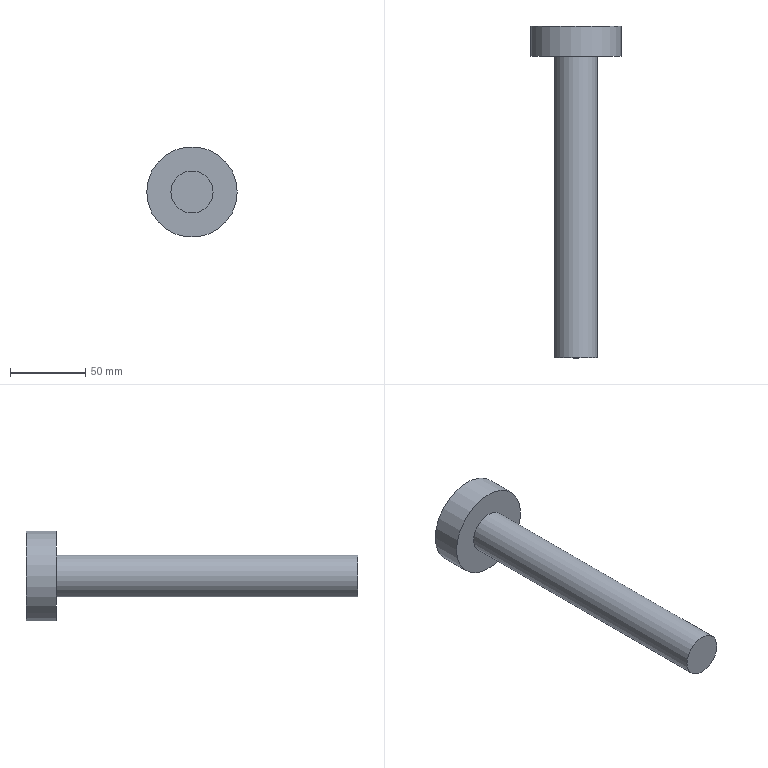Component | NX | PIN_2 | 1 solid | 5 faces | box 60 x 220 x 60 mm | volume 179699 mm3 | plane 3 | cylinder 2 | commonest cylinder face diameters 28 x1 60 x1
STEP:
#1=CARTESIAN_POINT('',(0.,0.,0.));
#2=DIRECTION('',(0.,0.,1.));
#3=DIRECTION('',(1.,0.,0.));
#4=AXIS2_PLACEMENT_3D('',#1,#2,#3);
#5=CARTESIAN_POINT('',(191.055,38.,82.998));
#6=VERTEX_POINT('',#5);
#7=CARTESIAN_POINT('',(177.055,38.,82.998));
#8=DIRECTION('',(0.,1.,0.));
#9=DIRECTION('',(1.,0.,0.));
#10=AXIS2_PLACEMENT_3D('',#7,#8,#9);
#11=CIRCLE('',#10,14.);
#12=CARTESIAN_POINT('',(177.055,38.,82.998));
#13=DIRECTION('',(0.,-1.,0.));
#14=DIRECTION('',(-1.,0.,0.));
#15=AXIS2_PLACEMENT_3D('',#12,#13,#14);
#16=PLANE('',#15);
#17=CARTESIAN_POINT('',(-14.,0.));
#18=CARTESIAN_POINT('',(-14.,24.249));
#19=CARTESIAN_POINT('',(7.,12.124));
#20=CARTESIAN_POINT('',(28.,0.));
#21=CARTESIAN_POINT('',(7.,-12.124));
#22=CARTESIAN_POINT('',(-14.,-24.249));
#23=CARTESIAN_POINT('',(-14.,0.));
#24=(BOUNDED_CURVE()B_SPLINE_CURVE(2,(#17,#18,#19,#20,#21,#22,#23),.UNSPECIFIED.,.T.,.F.)B_SPLINE_CURVE_WITH_KNOTS((1,2,2,2,2,1),(-2.094,0.,2.094,4.189,6.283,8.378),.UNSPECIFIED.)CURVE()GEOMETRIC_REPRESENTATION_ITEM()RATIONAL_B_SPLINE_CURVE((1.,0.5,1.,0.5,1.,0.5,1.))REPRESENTATION_ITEM(''));
#25=(GEOMETRIC_REPRESENTATION_CONTEXT(2)PARAMETRIC_REPRESENTATION_CONTEXT()REPRESENTATION_CONTEXT('',''));
#26=DEFINITIONAL_REPRESENTATION('',(#24),#25);
#27=PCURVE('',#16,#26);
#28=CARTESIAN_POINT('',(177.055,38.,82.998));
#29=DIRECTION('',(0.,1.,0.));
#30=DIRECTION('',(1.,0.,0.));
#31=AXIS2_PLACEMENT_3D('',#28,#29,#30);
#32=CYLINDRICAL_SURFACE('',#31,14.);
#33=CARTESIAN_POINT('',(0.,0.));
#34=DIRECTION('',(1.,0.));
#35=VECTOR('',#34,1.);
#36=LINE('',#33,#35);
#37=(GEOMETRIC_REPRESENTATION_CONTEXT(2)PARAMETRIC_REPRESENTATION_CONTEXT()REPRESENTATION_CONTEXT('',''));
#38=DEFINITIONAL_REPRESENTATION('',(#36),#37);
#39=PCURVE('',#32,#38);
#40=SURFACE_CURVE('',#11,(#27,#39),.PCURVE_S1.);
#41=EDGE_CURVE('',#6,#6,#40,.T.);
#42=ORIENTED_EDGE('',*,*,#41,.F.);
#43=EDGE_LOOP('',(#42));
#44=FACE_BOUND('',#43,.T.);
#45=ADVANCED_FACE('',(#44),#16,.T.);
#46=CARTESIAN_POINT('',(191.055,238.,82.998));
#47=VERTEX_POINT('',#46);
#48=CARTESIAN_POINT('',(177.055,238.,82.998));
#49=DIRECTION('',(0.,-1.,0.));
#50=DIRECTION('',(1.,0.,0.));
#51=AXIS2_PLACEMENT_3D('',#48,#49,#50);
#52=CIRCLE('',#51,14.);
#53=CARTESIAN_POINT('',(6.283,200.));
#54=DIRECTION('',(-1.,0.));
#55=VECTOR('',#54,1.);
#56=LINE('',#53,#55);
#57=(GEOMETRIC_REPRESENTATION_CONTEXT(2)PARAMETRIC_REPRESENTATION_CONTEXT()REPRESENTATION_CONTEXT('',''));
#58=DEFINITIONAL_REPRESENTATION('',(#56),#57);
#59=PCURVE('',#32,#58);
#60=CARTESIAN_POINT('',(177.055,238.,82.998));
#61=DIRECTION('',(0.,-1.,0.));
#62=DIRECTION('',(-1.,0.,0.));
#63=AXIS2_PLACEMENT_3D('',#60,#61,#62);
#64=PLANE('',#63);
#65=CARTESIAN_POINT('',(0.,0.));
#66=DIRECTION('',(-1.,0.));
#67=AXIS2_PLACEMENT_2D('',#65,#66);
#68=CIRCLE('',#67,14.);
#69=(GEOMETRIC_REPRESENTATION_CONTEXT(2)PARAMETRIC_REPRESENTATION_CONTEXT()REPRESENTATION_CONTEXT('',''));
#70=DEFINITIONAL_REPRESENTATION('',(#68),#69);
#71=PCURVE('',#64,#70);
#72=SURFACE_CURVE('',#52,(#59,#71),.PCURVE_S1.);
#73=EDGE_CURVE('',#47,#47,#72,.T.);
#74=ORIENTED_EDGE('',*,*,#73,.T.);
#75=CARTESIAN_POINT('',(191.055,38.,82.998));
#76=CARTESIAN_POINT('',(191.055,238.,82.998));
#77=B_SPLINE_CURVE_WITH_KNOTS('',1,(#75,#76),.UNSPECIFIED.,.F.,.F.,(2,2),(0.,200.),.PIECEWISE_BEZIER_KNOTS.);
#78=CARTESIAN_POINT('',(0.,0.));
#79=DIRECTION('',(0.,1.));
#80=VECTOR('',#79,1.);
#81=LINE('',#78,#80);
#82=(GEOMETRIC_REPRESENTATION_CONTEXT(2)PARAMETRIC_REPRESENTATION_CONTEXT()REPRESENTATION_CONTEXT('',''));
#83=DEFINITIONAL_REPRESENTATION('',(#81),#82);
#84=PCURVE('',#32,#83);
#85=CARTESIAN_POINT('',(6.283,0.));
#86=DIRECTION('',(0.,1.));
#87=VECTOR('',#86,1.);
#88=LINE('',#85,#87);
#89=(GEOMETRIC_REPRESENTATION_CONTEXT(2)PARAMETRIC_REPRESENTATION_CONTEXT()REPRESENTATION_CONTEXT('',''));
#90=DEFINITIONAL_REPRESENTATION('',(#88),#89);
#91=PCURVE('',#32,#90);
#92=SEAM_CURVE('',#77,(#84,#91),.PCURVE_S1.);
#93=EDGE_CURVE('',#6,#47,#92,.T.);
#94=ORIENTED_EDGE('',*,*,#93,.F.);
#95=ORIENTED_EDGE('',*,*,#41,.T.);
#96=ORIENTED_EDGE('',*,*,#93,.T.);
#97=EDGE_LOOP('',(#74,#94,#95,#96));
#98=FACE_BOUND('',#97,.T.);
#99=ADVANCED_FACE('',(#98),#32,.T.);
#100=CARTESIAN_POINT('',(207.055,258.,82.998));
#101=VERTEX_POINT('',#100);
#102=CARTESIAN_POINT('',(177.055,258.,82.998));
#103=DIRECTION('',(0.,-1.,0.));
#104=DIRECTION('',(1.,0.,0.));
#105=AXIS2_PLACEMENT_3D('',#102,#103,#104);
#106=CIRCLE('',#105,30.);
#107=CARTESIAN_POINT('',(177.055,258.,82.998));
#108=DIRECTION('',(0.,1.,0.));
#109=DIRECTION('',(1.,0.,0.));
#110=AXIS2_PLACEMENT_3D('',#107,#108,#109);
#111=PLANE('',#110);
#112=CARTESIAN_POINT('',(30.,0.));
#113=CARTESIAN_POINT('',(30.,-51.962));
#114=CARTESIAN_POINT('',(-15.,-25.981));
#115=CARTESIAN_POINT('',(-60.,-0.));
#116=CARTESIAN_POINT('',(-15.,25.981));
#117=CARTESIAN_POINT('',(30.,51.962));
#118=CARTESIAN_POINT('',(30.,0.));
#119=(BOUNDED_CURVE()B_SPLINE_CURVE(2,(#112,#113,#114,#115,#116,#117,#118),.UNSPECIFIED.,.T.,.F.)B_SPLINE_CURVE_WITH_KNOTS((1,2,2,2,2,1),(-2.094,0.,2.094,4.189,6.283,8.378),.UNSPECIFIED.)CURVE()GEOMETRIC_REPRESENTATION_ITEM()RATIONAL_B_SPLINE_CURVE((1.,0.5,1.,0.5,1.,0.5,1.))REPRESENTATION_ITEM(''));
#120=(GEOMETRIC_REPRESENTATION_CONTEXT(2)PARAMETRIC_REPRESENTATION_CONTEXT()REPRESENTATION_CONTEXT('',''));
#121=DEFINITIONAL_REPRESENTATION('',(#119),#120);
#122=PCURVE('',#111,#121);
#123=CARTESIAN_POINT('',(177.055,238.,82.998));
#124=DIRECTION('',(0.,1.,0.));
#125=DIRECTION('',(1.,0.,0.));
#126=AXIS2_PLACEMENT_3D('',#123,#124,#125);
#127=CYLINDRICAL_SURFACE('',#126,30.);
#128=CARTESIAN_POINT('',(6.283,20.));
#129=DIRECTION('',(-1.,0.));
#130=VECTOR('',#129,1.);
#131=LINE('',#128,#130);
#132=(GEOMETRIC_REPRESENTATION_CONTEXT(2)PARAMETRIC_REPRESENTATION_CONTEXT()REPRESENTATION_CONTEXT('',''));
#133=DEFINITIONAL_REPRESENTATION('',(#131),#132);
#134=PCURVE('',#127,#133);
#135=SURFACE_CURVE('',#106,(#122,#134),.PCURVE_S1.);
#136=EDGE_CURVE('',#101,#101,#135,.T.);
#137=ORIENTED_EDGE('',*,*,#136,.F.);
#138=EDGE_LOOP('',(#137));
#139=FACE_BOUND('',#138,.T.);
#140=ADVANCED_FACE('',(#139),#111,.T.);
#141=ORIENTED_EDGE('',*,*,#73,.F.);
#142=EDGE_LOOP('',(#141));
#143=FACE_BOUND('',#142,.T.);
#144=CARTESIAN_POINT('',(207.055,238.,82.998));
#145=VERTEX_POINT('',#144);
#146=CARTESIAN_POINT('',(177.055,238.,82.998));
#147=DIRECTION('',(0.,1.,0.));
#148=DIRECTION('',(1.,0.,0.));
#149=AXIS2_PLACEMENT_3D('',#146,#147,#148);
#150=CIRCLE('',#149,30.);
#151=CARTESIAN_POINT('',(-30.,0.));
#152=CARTESIAN_POINT('',(-30.,51.962));
#153=CARTESIAN_POINT('',(15.,25.981));
#154=CARTESIAN_POINT('',(60.,0.));
#155=CARTESIAN_POINT('',(15.,-25.981));
#156=CARTESIAN_POINT('',(-30.,-51.962));
#157=CARTESIAN_POINT('',(-30.,0.));
#158=(BOUNDED_CURVE()B_SPLINE_CURVE(2,(#151,#152,#153,#154,#155,#156,#157),.UNSPECIFIED.,.T.,.F.)B_SPLINE_CURVE_WITH_KNOTS((1,2,2,2,2,1),(-2.094,0.,2.094,4.189,6.283,8.378),.UNSPECIFIED.)CURVE()GEOMETRIC_REPRESENTATION_ITEM()RATIONAL_B_SPLINE_CURVE((1.,0.5,1.,0.5,1.,0.5,1.))REPRESENTATION_ITEM(''));
#159=(GEOMETRIC_REPRESENTATION_CONTEXT(2)PARAMETRIC_REPRESENTATION_CONTEXT()REPRESENTATION_CONTEXT('',''));
#160=DEFINITIONAL_REPRESENTATION('',(#158),#159);
#161=PCURVE('',#64,#160);
#162=CARTESIAN_POINT('',(0.,0.));
#163=DIRECTION('',(1.,0.));
#164=VECTOR('',#163,1.);
#165=LINE('',#162,#164);
#166=(GEOMETRIC_REPRESENTATION_CONTEXT(2)PARAMETRIC_REPRESENTATION_CONTEXT()REPRESENTATION_CONTEXT('',''));
#167=DEFINITIONAL_REPRESENTATION('',(#165),#166);
#168=PCURVE('',#127,#167);
#169=SURFACE_CURVE('',#150,(#161,#168),.PCURVE_S1.);
#170=EDGE_CURVE('',#145,#145,#169,.T.);
#171=ORIENTED_EDGE('',*,*,#170,.F.);
#172=EDGE_LOOP('',(#171));
#173=FACE_BOUND('',#172,.T.);
#174=ADVANCED_FACE('',(#143,#173),#64,.T.);
#175=ORIENTED_EDGE('',*,*,#136,.T.);
#176=CARTESIAN_POINT('',(207.055,238.,82.998));
#177=CARTESIAN_POINT('',(207.055,258.,82.998));
#178=B_SPLINE_CURVE_WITH_KNOTS('',1,(#176,#177),.UNSPECIFIED.,.F.,.F.,(2,2),(0.,20.),.PIECEWISE_BEZIER_KNOTS.);
#179=CARTESIAN_POINT('',(0.,0.));
#180=DIRECTION('',(0.,1.));
#181=VECTOR('',#180,1.);
#182=LINE('',#179,#181);
#183=(GEOMETRIC_REPRESENTATION_CONTEXT(2)PARAMETRIC_REPRESENTATION_CONTEXT()REPRESENTATION_CONTEXT('',''));
#184=DEFINITIONAL_REPRESENTATION('',(#182),#183);
#185=PCURVE('',#127,#184);
#186=CARTESIAN_POINT('',(6.283,0.));
#187=DIRECTION('',(0.,1.));
#188=VECTOR('',#187,1.);
#189=LINE('',#186,#188);
#190=(GEOMETRIC_REPRESENTATION_CONTEXT(2)PARAMETRIC_REPRESENTATION_CONTEXT()REPRESENTATION_CONTEXT('',''));
#191=DEFINITIONAL_REPRESENTATION('',(#189),#190);
#192=PCURVE('',#127,#191);
#193=SEAM_CURVE('',#178,(#185,#192),.PCURVE_S1.);
#194=EDGE_CURVE('',#145,#101,#193,.T.);
#195=ORIENTED_EDGE('',*,*,#194,.F.);
#196=ORIENTED_EDGE('',*,*,#170,.T.);
#197=ORIENTED_EDGE('',*,*,#194,.T.);
#198=EDGE_LOOP('',(#175,#195,#196,#197));
#199=FACE_BOUND('',#198,.T.);
#200=ADVANCED_FACE('',(#199),#127,.T.);
#201=CLOSED_SHELL('',(#45,#99,#140,#174,#200));
#202=MANIFOLD_SOLID_BREP('',#201);
#203=(LENGTH_UNIT()NAMED_UNIT(*)SI_UNIT(.MILLI.,.METRE.));
#204=UNCERTAINTY_MEASURE_WITH_UNIT(LENGTH_MEASURE(0.00001),#203,'','');
#205=(NAMED_UNIT(*)PLANE_ANGLE_UNIT()SI_UNIT($,.RADIAN.));
#206=(NAMED_UNIT(*)SI_UNIT($,.STERADIAN.)SOLID_ANGLE_UNIT());
#207=(GEOMETRIC_REPRESENTATION_CONTEXT(3)GLOBAL_UNCERTAINTY_ASSIGNED_CONTEXT((#204))GLOBAL_UNIT_ASSIGNED_CONTEXT((#203,#205,#206))REPRESENTATION_CONTEXT('',''));
#208=ADVANCED_BREP_SHAPE_REPRESENTATION('',(#4,#202),#207);